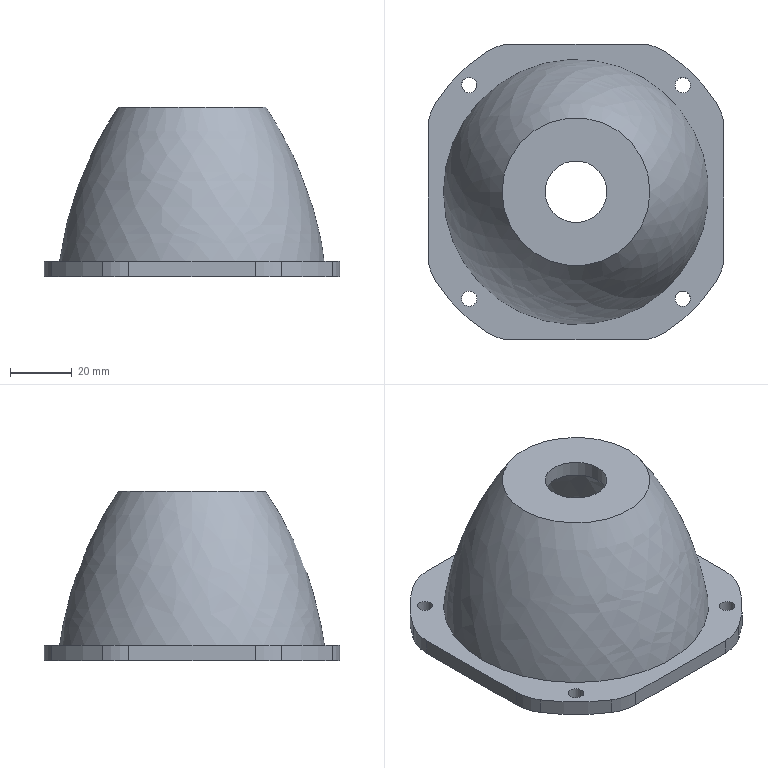Component | NX | TOP_COVER | 1 solid | 27 faces | volume 81612 mm3 | cylinder 17 | plane 8 | spline 2 | commonest cylinder face diameters 32 x8 108 x4 5 x4 20 x1